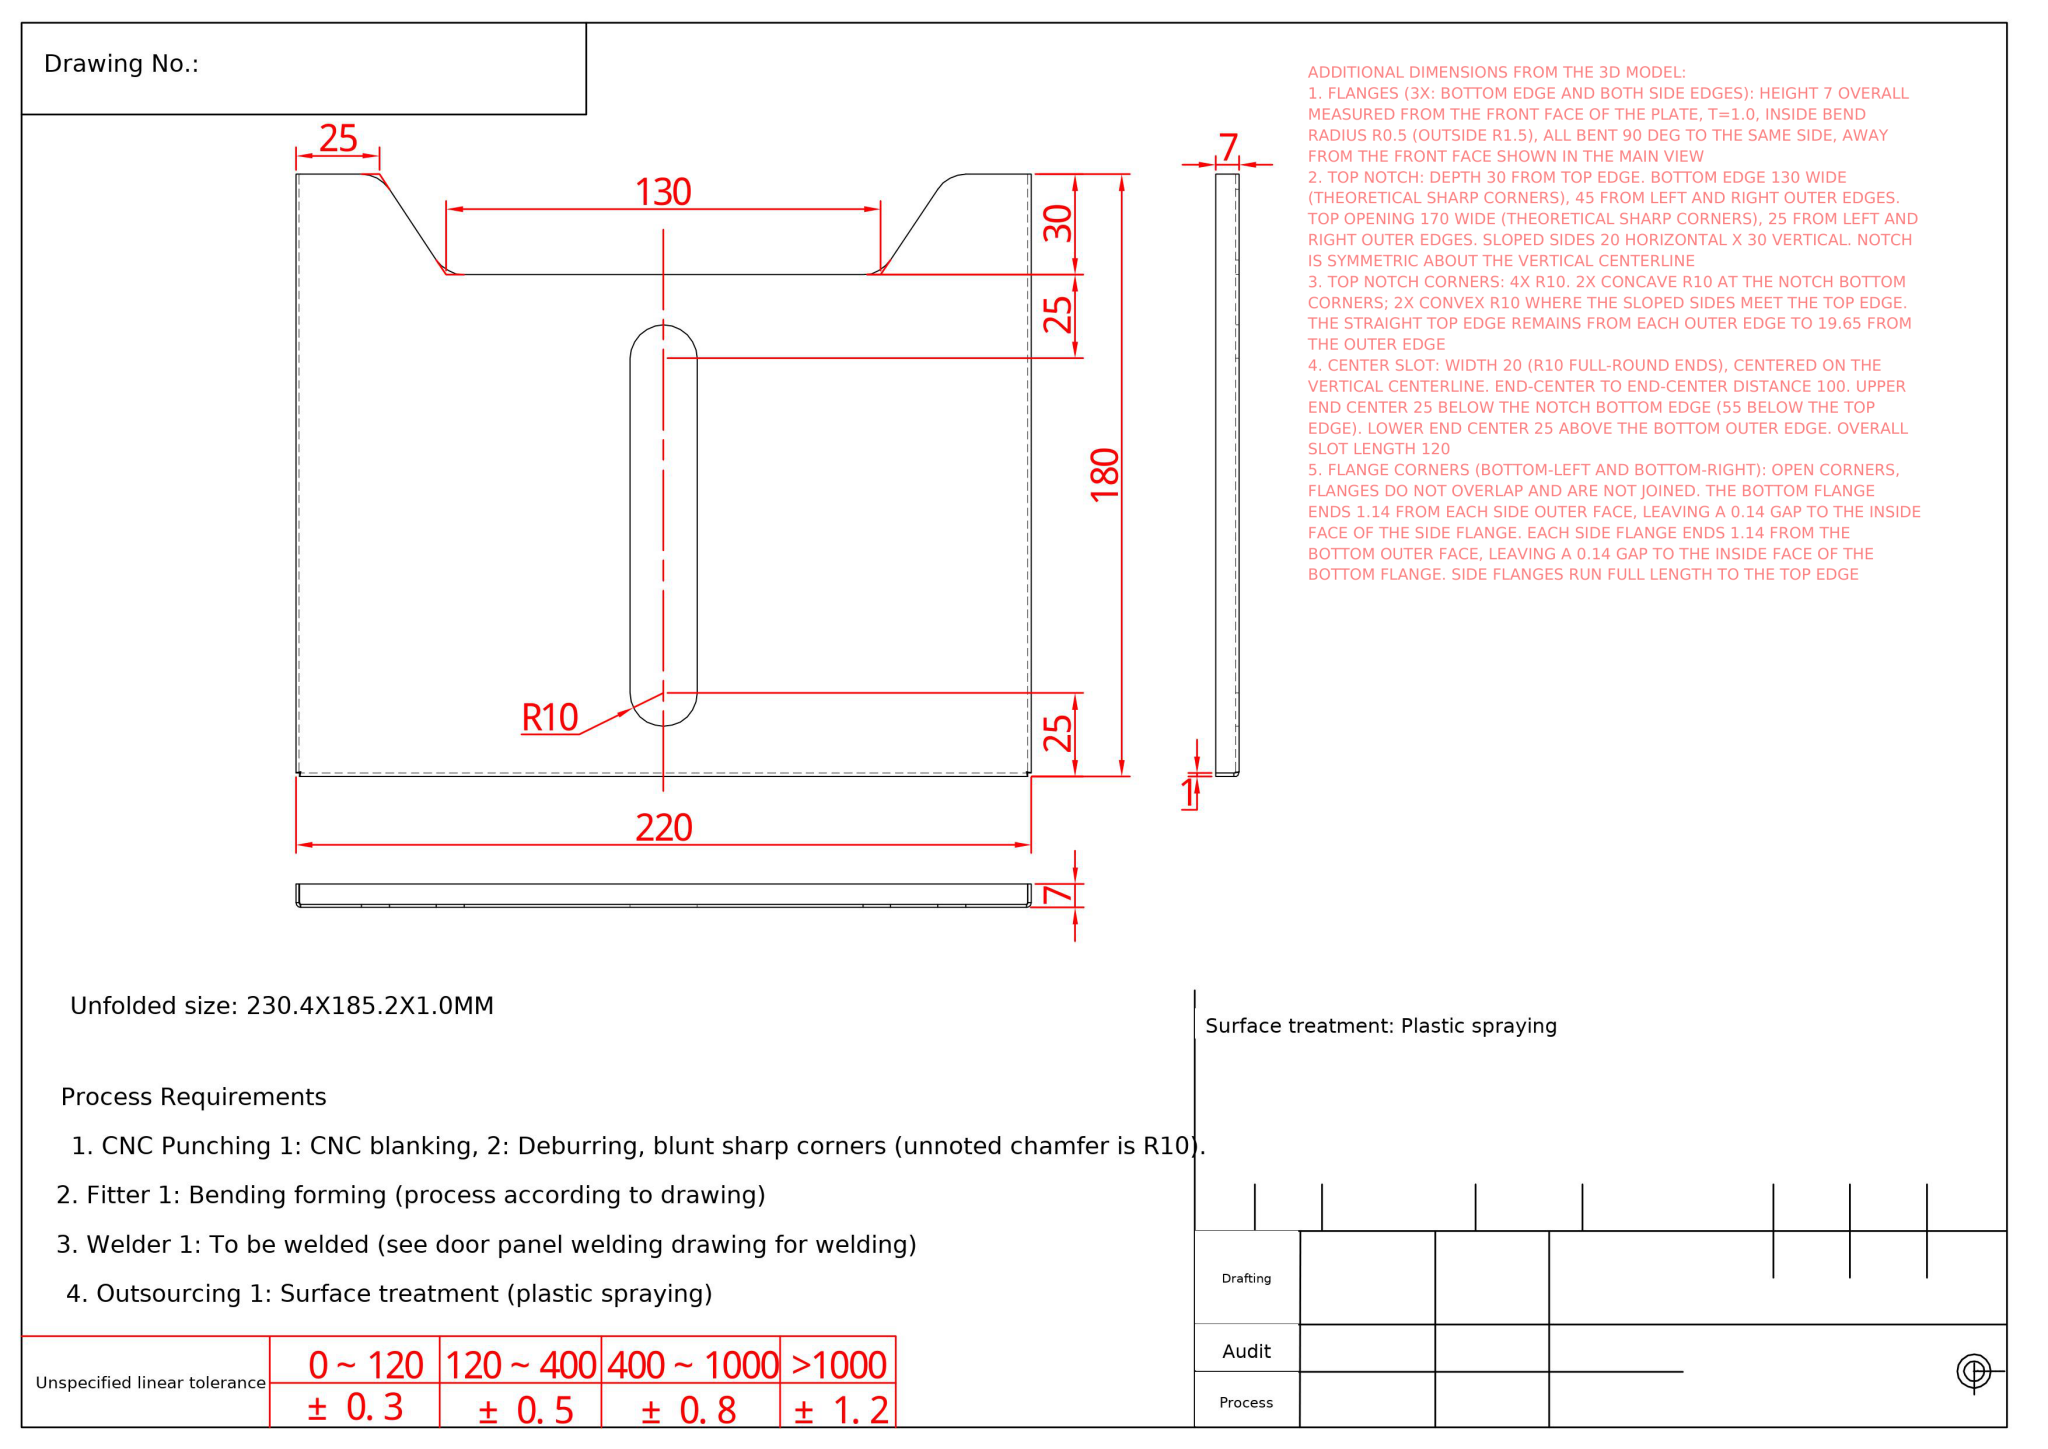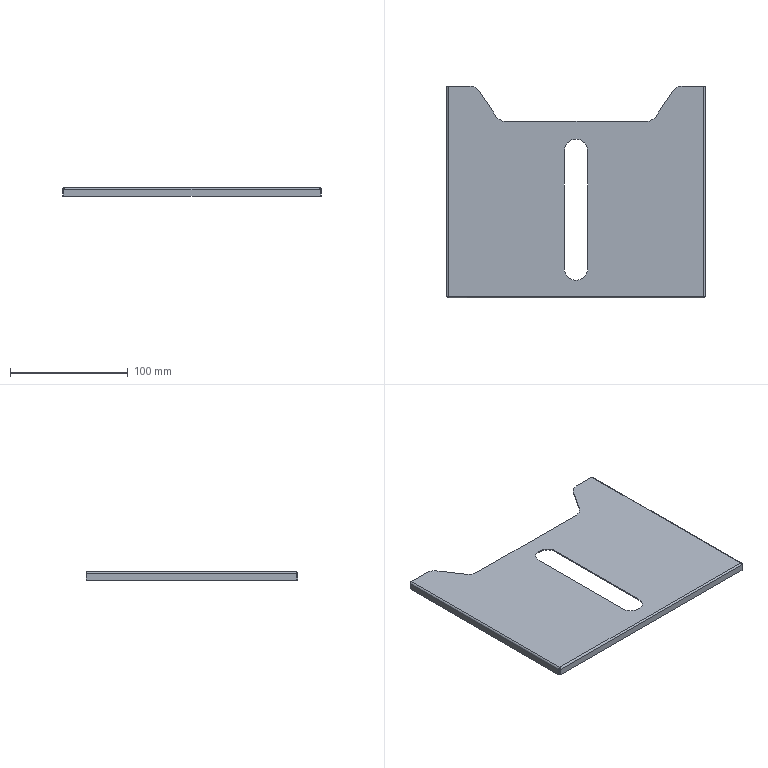Part | NX | mm | 1 solid | 42 faces | box 220 x 180 x 7 mm | volume 35988 mm3 | plane 26 | cylinder 12 | spline 4 | commonest cylinder face diameters 20 x6 3 x3 1 x3